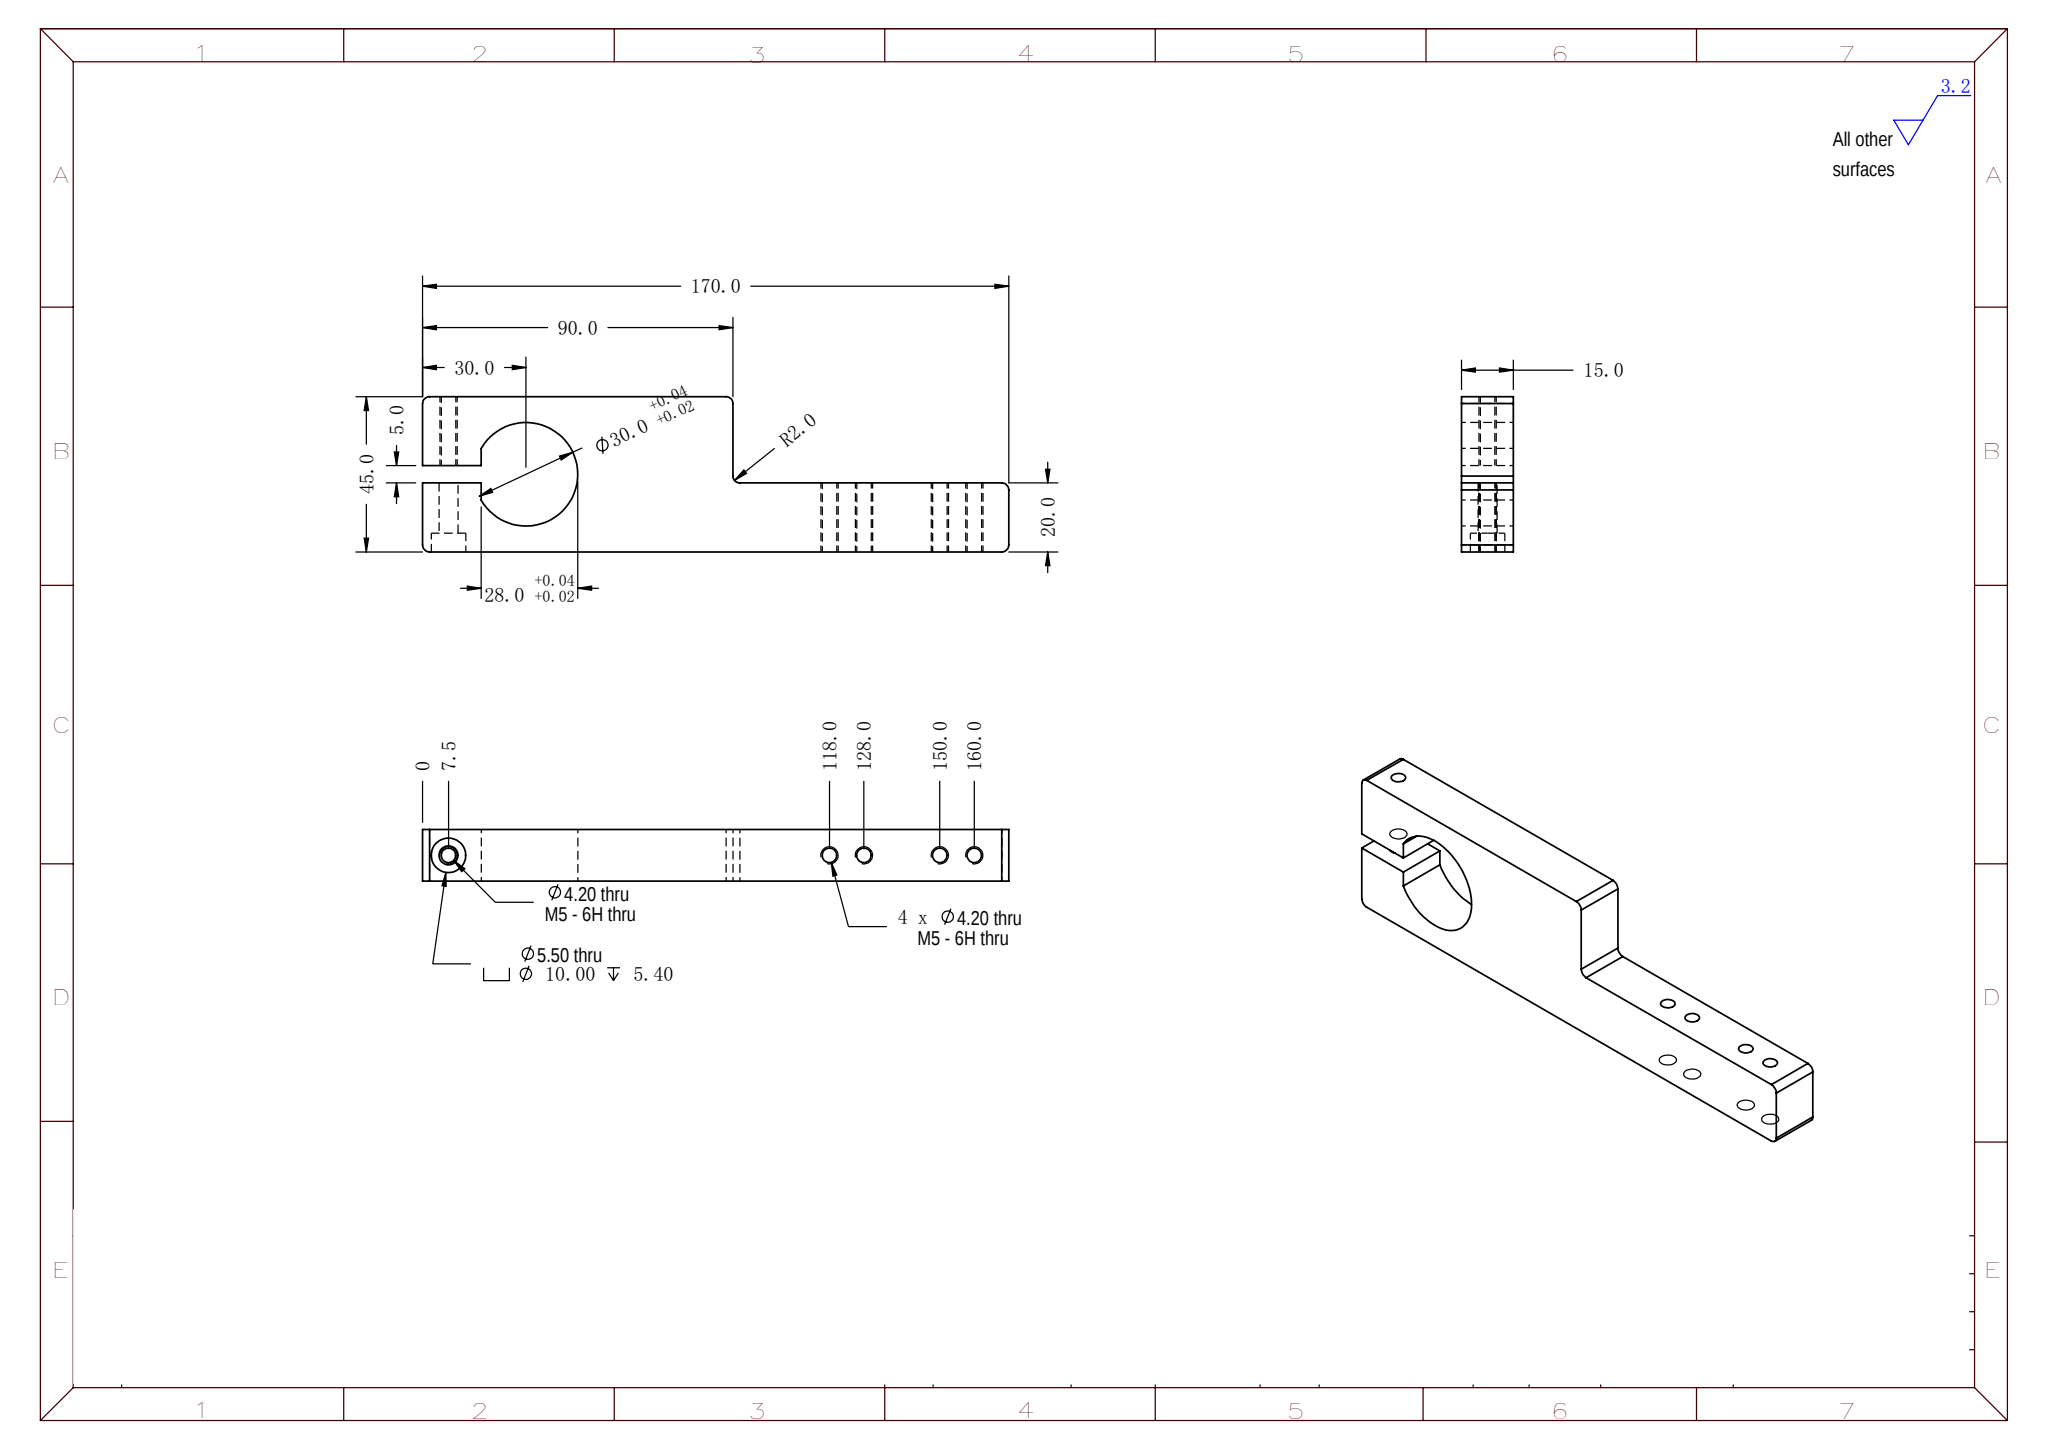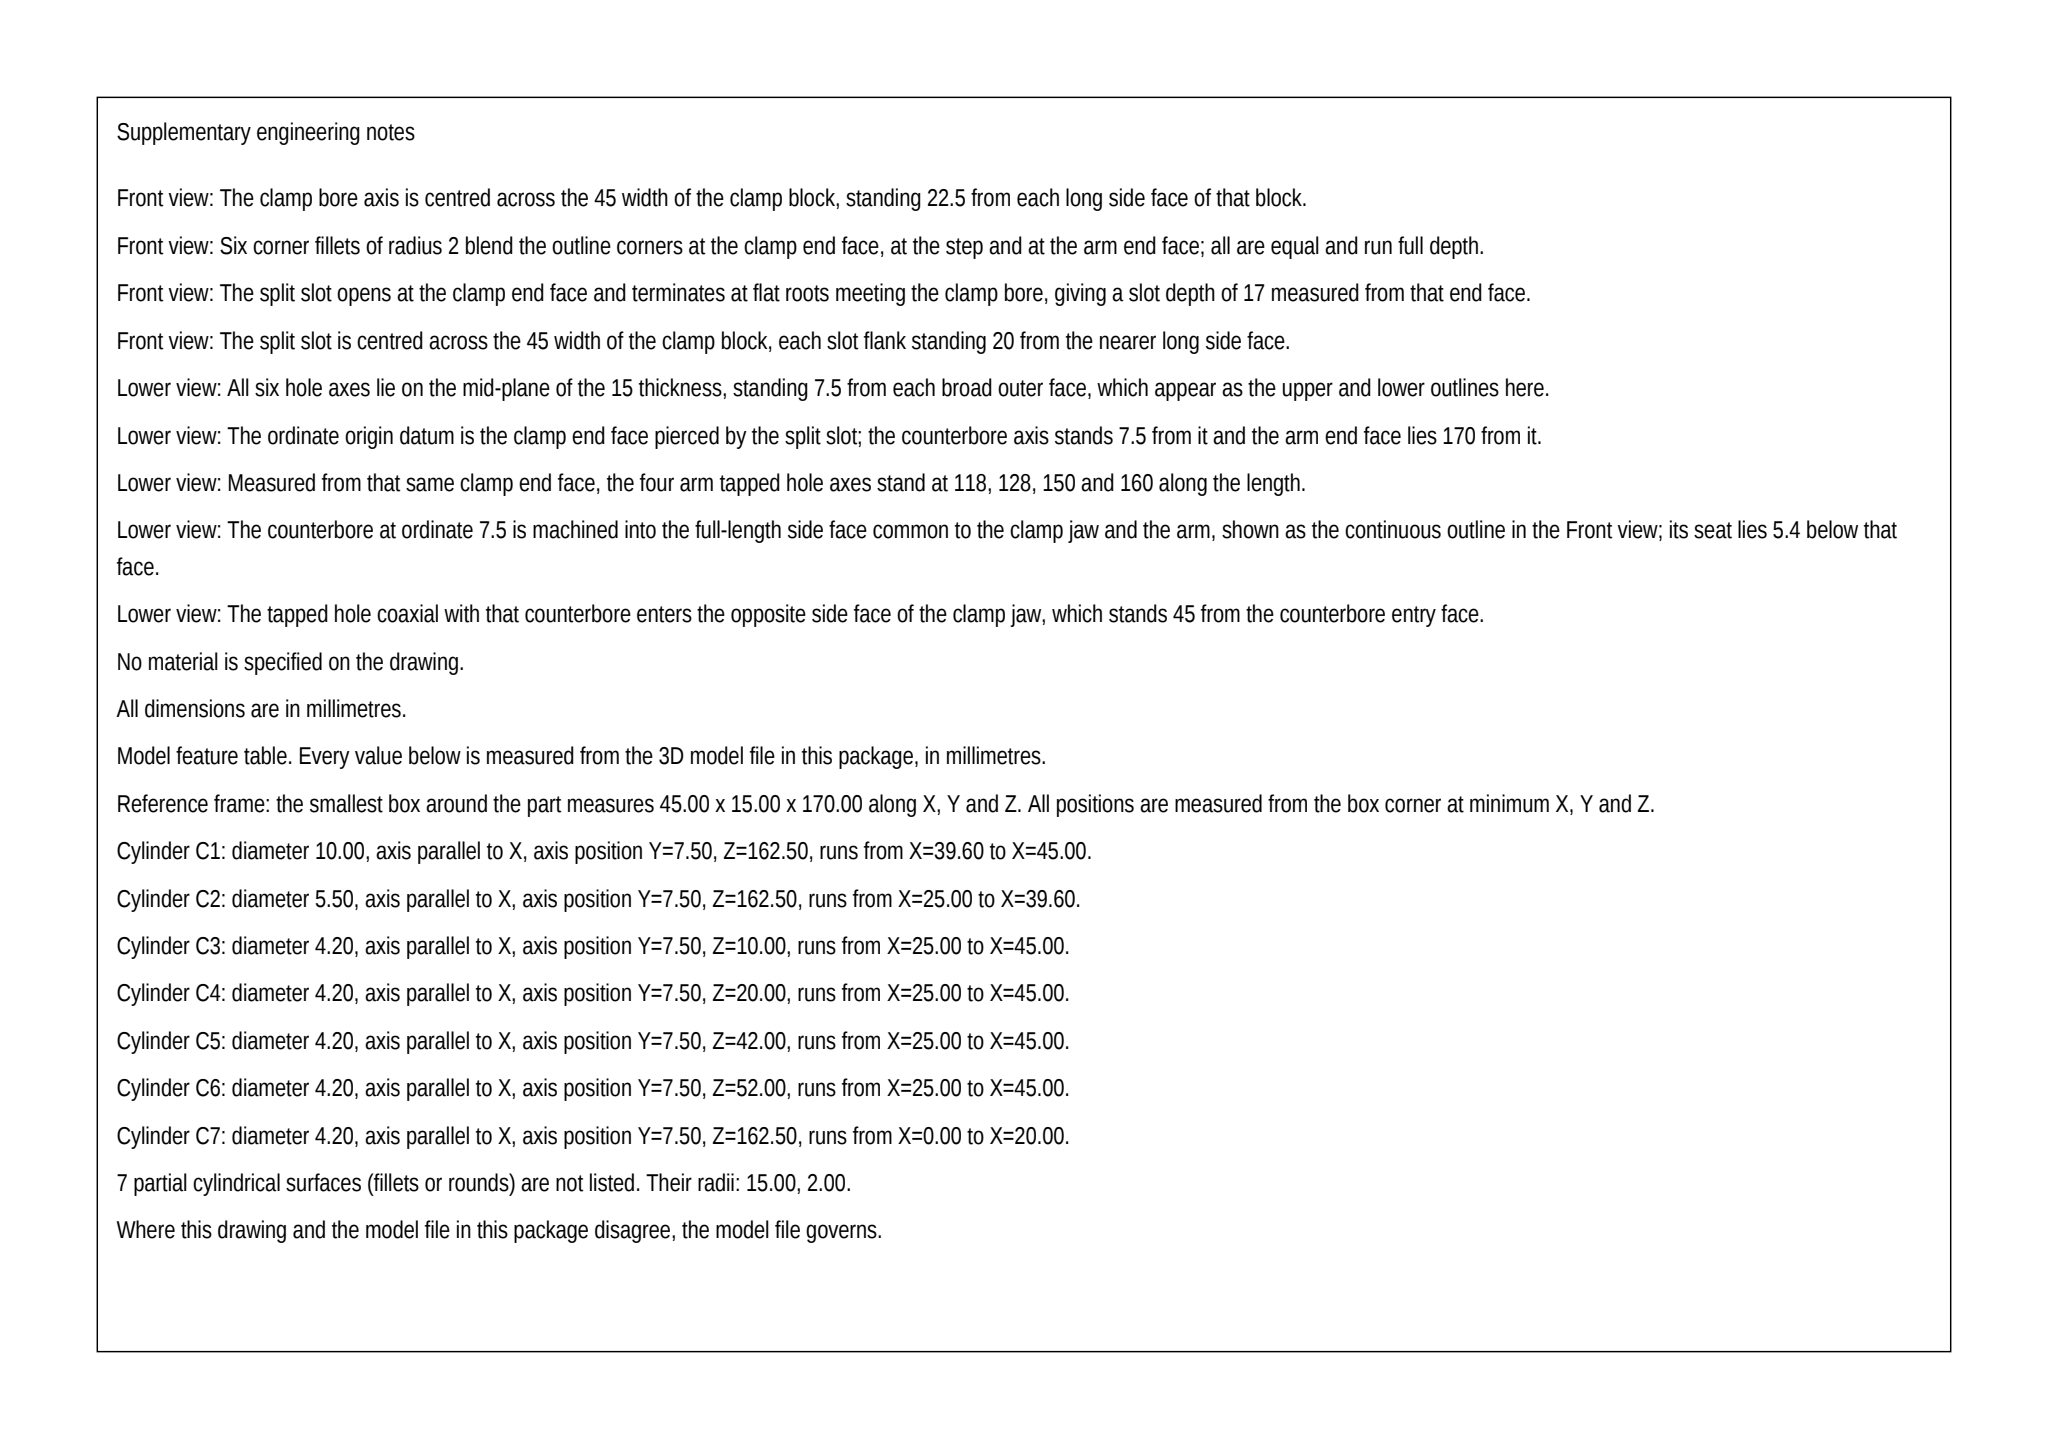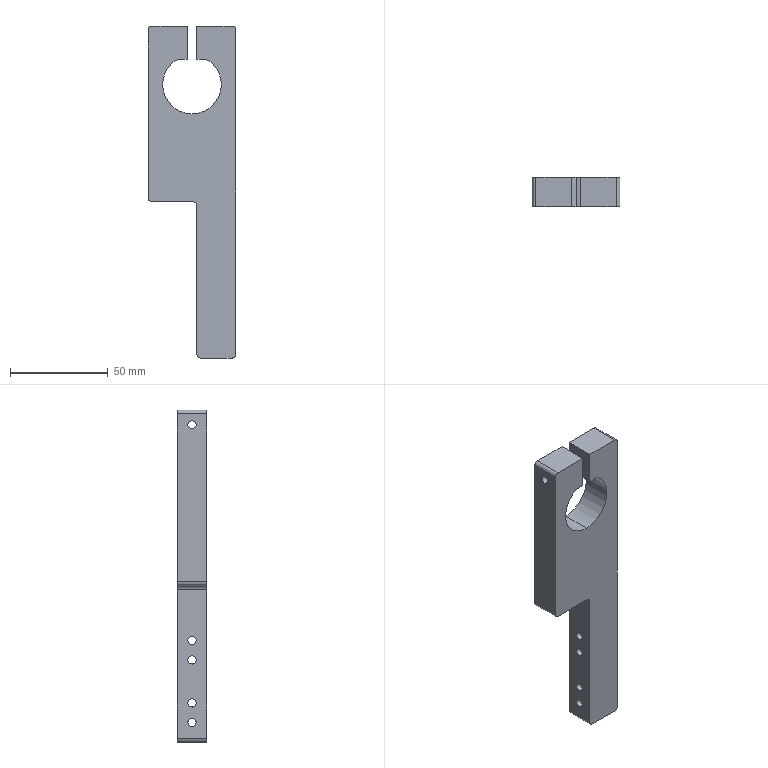Part | SolidWorks | mm | 1 solid | 36 faces | box 45 x 15 x 170 mm | volume 70968 mm3 | cylinder 22 | plane 14 | commonest cylinder face diameters 4.2 x10 4 x6 10 x2 5.5 x2 30 x2
Drawing notes:
Ø30 BORE AXIS & 5.0 SLIT C/L AT 22.5 FROM EACH 45.0 FACE | from the solid: Slit faces x=20 & x=25 (5.0 wide); Ø30 cyl axis at x=22.5 in 45.0 bbox
ALL Ø4.20/M5 & Ø5.50-Ø10.00 HOLES ON C/L 7.5 FROM EACH FACE | from the solid: All x-axis holes (Ø4.2, Ø5.5, Ø10) at y=7.5 of 15.0 thk
ALL ROUNDED CORNERS R2.0 TYP | from the solid: Ø4.0 y-axis corner cyls at (2,82),(2,168),(23,78),(27,2),(43,2),(43,168)
build123d program:
from build123d import *

# Parameters (mm, degrees)
BOSS_EXTRUDE1_DEPTH                             = 7.5
M5_HEX_SOCKET_HEAD_CAP_SCREW_CBORE1_D           = 5.5
M5_HEX_SOCKET_HEAD_CAP_SCREW_CBORE1_DEPTH       = 20
M5_HEX_SOCKET_HEAD_CAP_SCREW_CBORE1_CBORE_D     = 10
M5_HEX_SOCKET_HEAD_CAP_SCREW_CBORE1_CBORE_DEPTH = 5.4
M5_TAPPED_HOLE1_D                               = 4.2
CUT_EXTRUDE1_REACH                              = 91.198
SKETCH8_W                                       = 25
SKETCH8_H                                       = 80
FILLET1_R                                       = 2
M5_TAPPED_HOLE2_D                               = 4.2


with BuildPart() as part:
    # Sketch1 → Boss-Extrude1 (new, symmetric)
    with BuildSketch(Plane(origin=(0, 0, 0), x_dir=(1, 0, 0), z_dir=(0, 1, 0))):
        with BuildLine():
            Line((-7.483, -68), (-2.5, -68))
            Line((-2.5, -68), (-2.5, -85))
            Line((-2.5, -85), (-22.5, -85))
            Line((-22.5, -85), (-22.5, 85))
            Line((-22.5, 85), (22.5, 85))
            Line((22.5, 85), (22.5, -85))
            Line((22.5, -85), (2.5, -85))
            Line((2.5, -85), (2.5, -68))
            Line((2.5, -68), (7.483, -68))
            ThreePointArc((7.483, -68), (0, -40), (-7.483, -68))
        make_face()
    extrude(amount=BOSS_EXTRUDE1_DEPTH, both=True)

    # M5 Hex Socket Head Cap Screw CBORE1
    with Locations(Plane(origin=(22.5, 0, 0), x_dir=(0, 0, -1), z_dir=(1, 0, 0))):
        with Locations((-77.5, 0)):
            CounterBoreHole(M5_HEX_SOCKET_HEAD_CAP_SCREW_CBORE1_D / 2, M5_HEX_SOCKET_HEAD_CAP_SCREW_CBORE1_CBORE_D / 2, M5_HEX_SOCKET_HEAD_CAP_SCREW_CBORE1_CBORE_DEPTH, depth=M5_HEX_SOCKET_HEAD_CAP_SCREW_CBORE1_DEPTH)

    # M5 Tapped Hole1 (through all)
    with Locations(Plane(origin=(-2.5, 0, 0), x_dir=(0, 0, -1), z_dir=(1, 0, 0))):
        with Locations((-77.5, 0)):
            Hole(M5_TAPPED_HOLE1_D / 2)

    # Sketch8 → Cut-Extrude1 (cut, up to next)
    with BuildSketch(Plane(origin=(0, 7.5, 0), x_dir=(1, 0, 0), z_dir=(0, 1, 0)), mode=Mode.PRIVATE) as cut_extrude1_sk1:
        with Locations((-10, 45)):
            Rectangle(SKETCH8_W, SKETCH8_H)
    cut_extrude1_tool1 = extrude(cut_extrude1_sk1.sketch, amount=-CUT_EXTRUDE1_REACH, mode=Mode.PRIVATE) & part.part
    add(cut_extrude1_tool1.solids().sort_by_distance((-10, 7.5, -45))[0], mode=Mode.SUBTRACT)

    # Fillet1
    fillet1_edges = [part.edges().sort_by_distance(p)[0] for p in [
        (22.5, 0, -85),
        (22.5, 0, 85),
        (-22.5, 0, 85),
        (-22.5, 0, -5),
        (2.5, 0, -85),
        (2.5, 0, -5),
    ]]
    fillet(fillet1_edges, radius=FILLET1_R)

    # M5 Tapped Hole2 (through all)
    with Locations(Plane(origin=(22.5, 0, 0), x_dir=(0, 0, -1), z_dir=(1, 0, 0))):
        with Locations((43, 0), (75, 0), (65, 0), (33, 0)):
            Hole(M5_TAPPED_HOLE2_D / 2)


solid = part.part